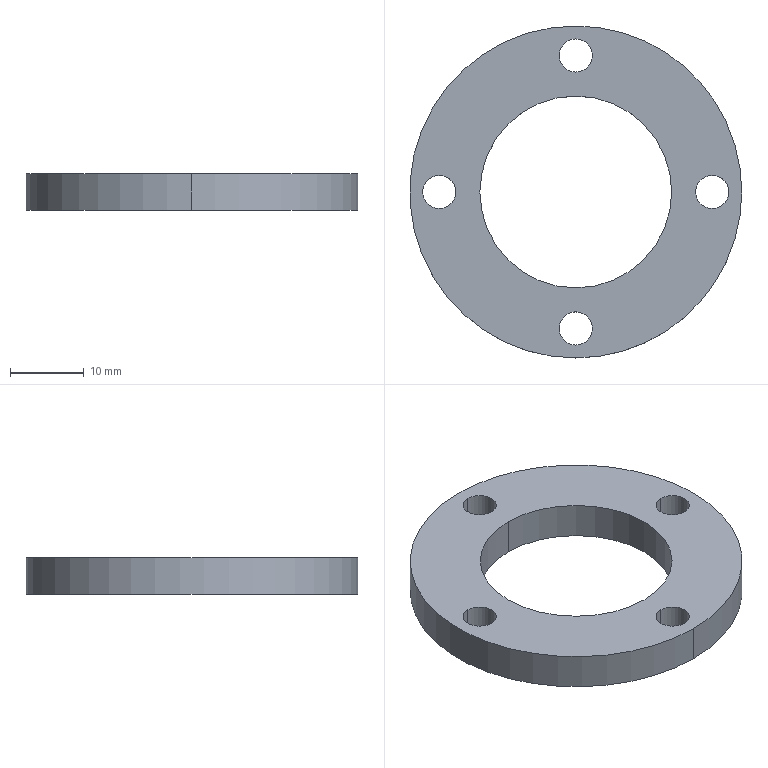CAM job | Mastercam | mm | 1 operations | part box 45 x 45 x 5
1. Drill/Counterbore | 7 - 4 倒角刀